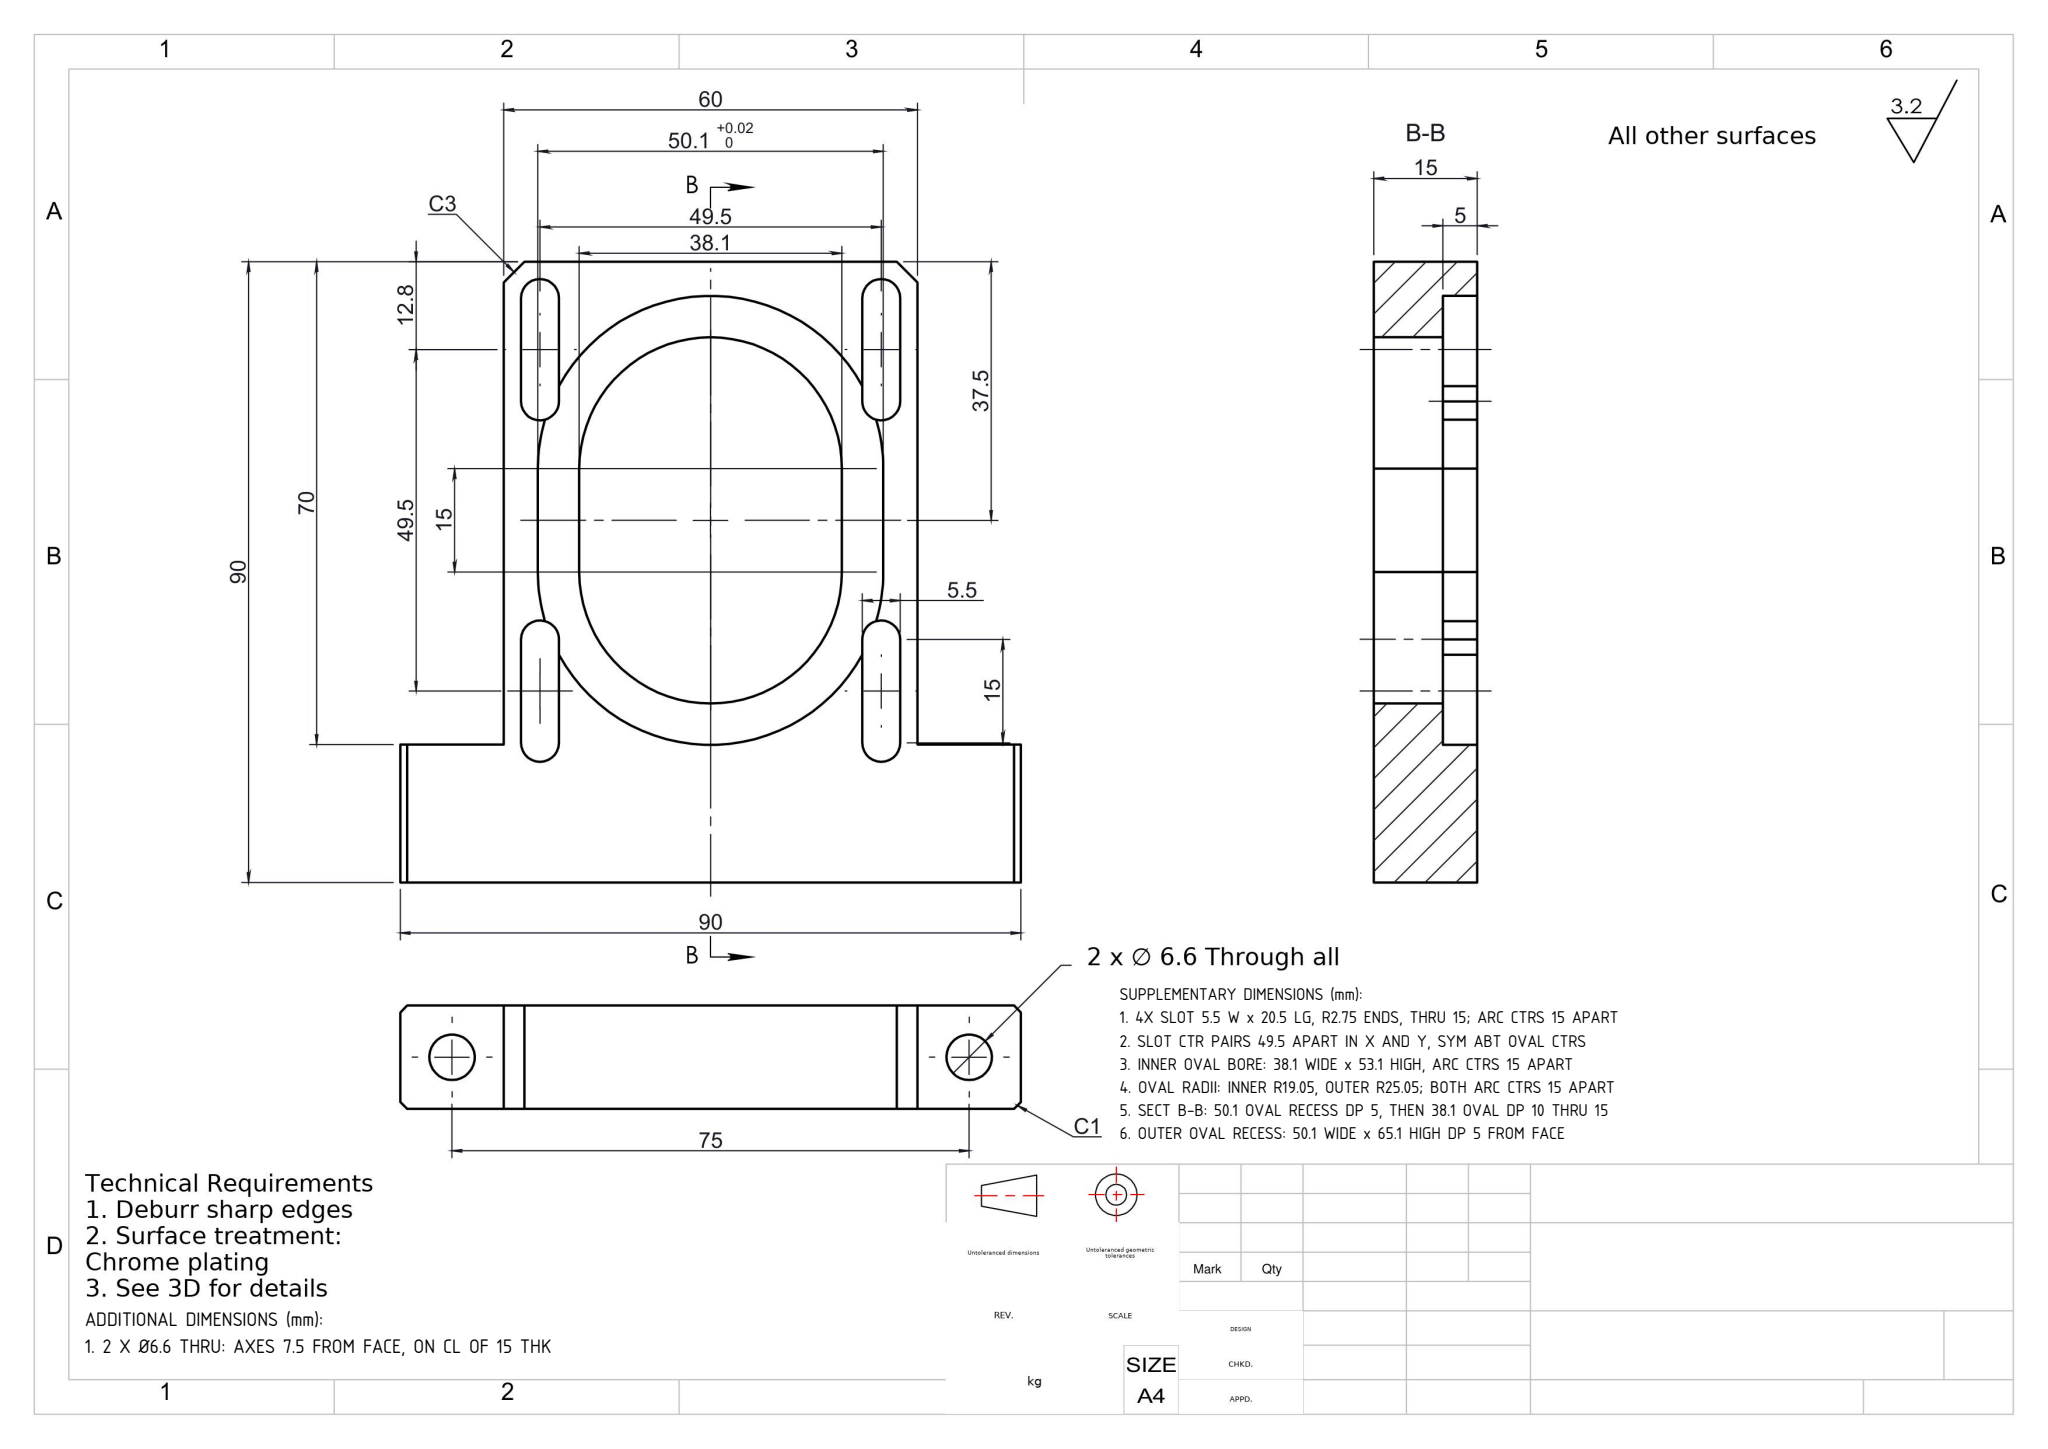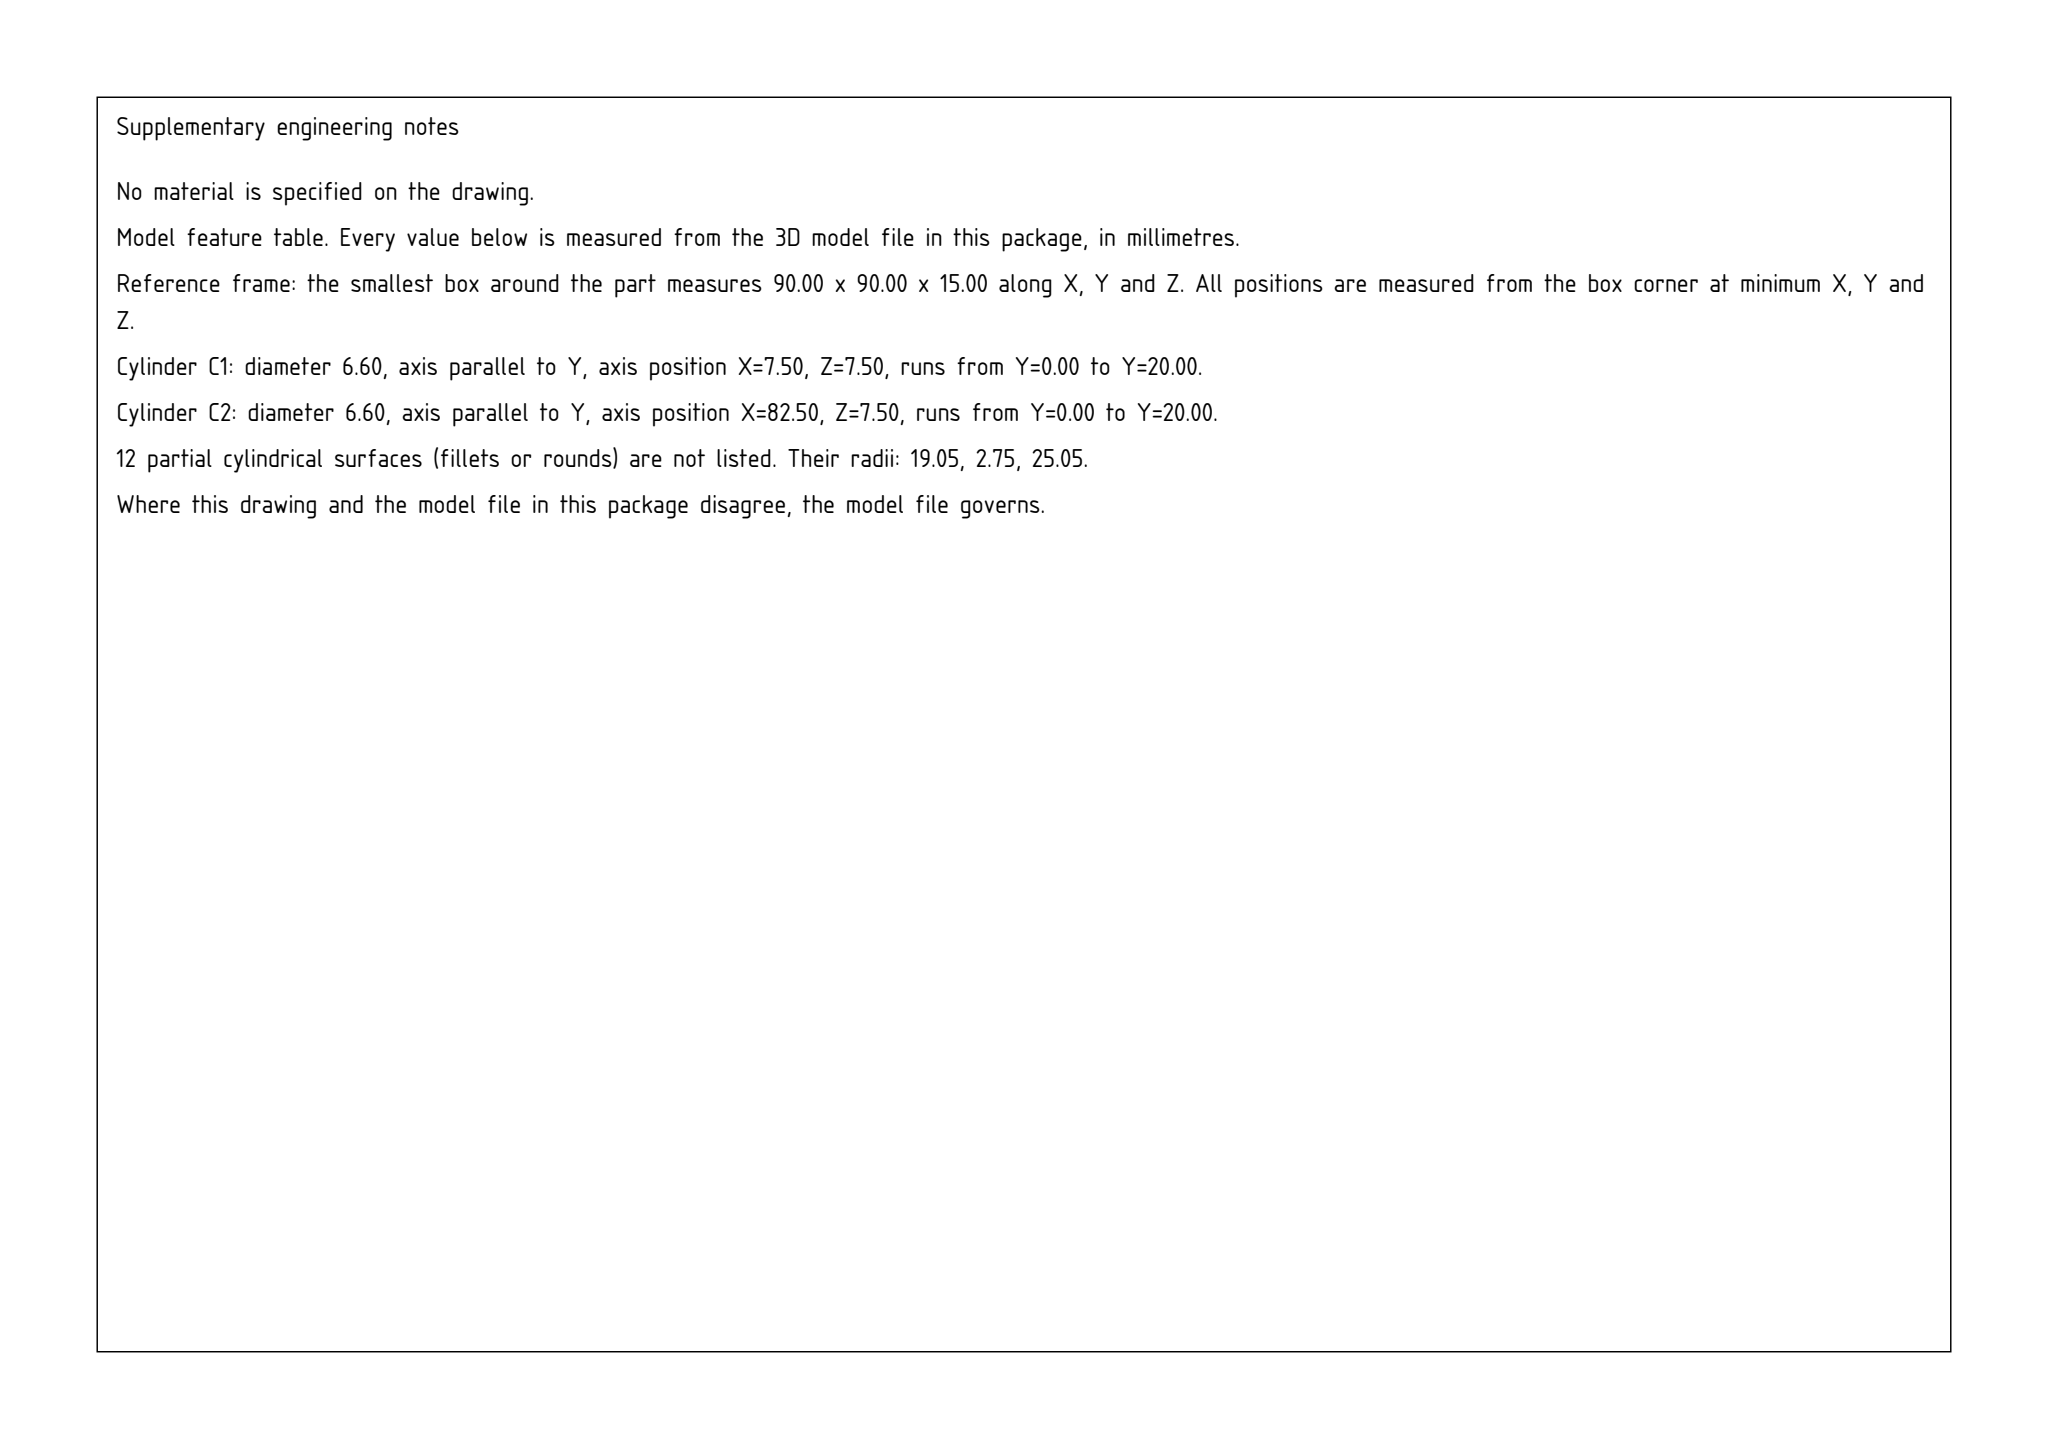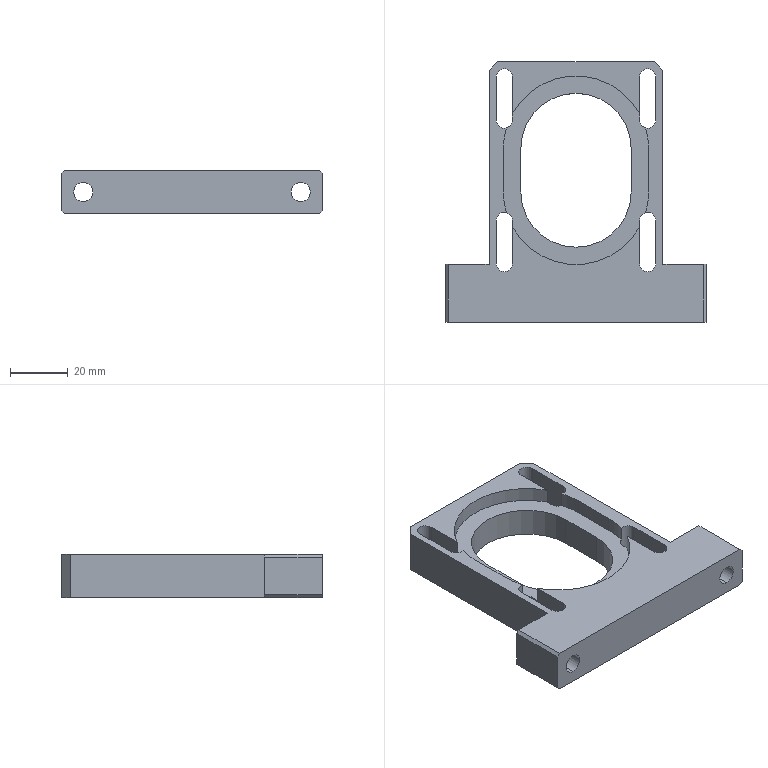Part | SolidWorks | mm | 1 solid | 49 faces | box 90 x 90 x 15 mm | volume 51431 mm3 | plane 29 | cylinder 20 | commonest cylinder face diameters 5.5 x8 50.1 x6 6.6 x4 38.1 x2